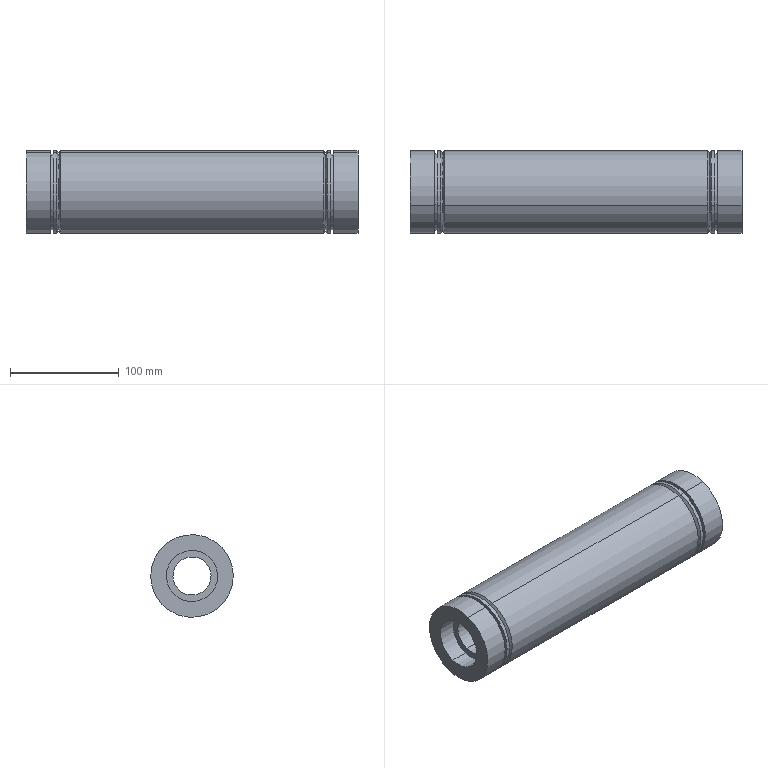Component | SolidWorks | DrivenRoller-1 | 3 solids | 50 faces | box 305 x 76 x 76 mm | volume 436807 mm3 | cylinder 28 | plane 14 | cone 8 | commonest cylinder face diameters 76 x10 68 x6 47 x4 35 x4 70 x4
build123d program:
from build123d import *
from OCP.BRepFilletAPI import BRepFilletAPI_MakeChamfer

# Parameters (mm, degrees)
SKETCH1_W      = 245
SKETCH1_H      = 4
CHAMFER1_SIZE  = 3
CHAMFER1_SIZE2 = 1.732
CHAMFER2_SIZE  = 3
CHAMFER2_SIZE2 = 1.732
CHAMFER3_SIZE  = 3
CHAMFER3_SIZE2 = 1.732


with BuildPart() as part:
    # Sketch1 → Revolve1 (revolve)
    with BuildSketch(Plane.XY, mode=Mode.PRIVATE) as revolve1_sk:
        with Locations((152.5, 36)):
            Rectangle(SKETCH1_W, SKETCH1_H)
    revolve(revolve1_sk.sketch.rotate(Axis((-4310.875, 0, 0), (1, 0, 0)), 90), axis=Axis((-4310.875, 0, 0), (1, 0, 0)))

    # Chamfer1: one chamfer whose edges measure the first distance from different faces: ONE call of the kernel's chamfer builder (chamfer() names one face for all edges)
    chamfer1_edges_1 = [part.edges().sort_by_distance(p)[0] for p in [
        (30, 0, -38),
    ]]
    chamfer1_side_1 = [part.faces().sort_by_distance(p)[0] for p in [
        (30, 0, -36.925),
    ]]
    chamfer1_edges_2 = [part.edges().sort_by_distance(p)[0] for p in [
        (275, 0, -38),
    ]]
    chamfer1_side_2 = [part.faces().sort_by_distance(p)[0] for p in [
        (275, 0, -35.075),
    ]]
    chamfer1 = BRepFilletAPI_MakeChamfer(part.part.solid().wrapped)
    for e in chamfer1_edges_1:
        chamfer1.Add(CHAMFER1_SIZE, CHAMFER1_SIZE2, e.wrapped, chamfer1_side_1[0].wrapped)  # the first distance lies on this face
    for e in chamfer1_edges_2:
        chamfer1.Add(CHAMFER1_SIZE, CHAMFER1_SIZE2, e.wrapped, chamfer1_side_2[0].wrapped)  # the first distance lies on this face
    add(Compound.cast(chamfer1.Shape()), mode=Mode.REPLACE)


with BuildPart() as body_2:
    # Sketch2 → Revolve2 (revolve)
    with BuildSketch(Plane.XY, mode=Mode.PRIVATE) as revolve2_sk:
        Polygon((0, 38), (22.5, 38), (22.5, 35), (25, 35), (25, 38), (30, 38), (30, 34), (36, 34), (36, 17.5), (16.5, 17.5), (16.5, 23.5), (0, 23.5), align=None)
        Polygon((275, 38), (280, 38), (280, 35), (282.5, 35), (282.5, 38), (305, 38), (305, 23.5), (288.5, 23.5), (288.5, 17.5), (269, 17.5), (269, 34), (275, 34), align=None)
    revolve(revolve2_sk.sketch.rotate(Axis((-1000, 0, 0), (1, 0, 0)), 90), axis=Axis((-1000, 0, 0), (1, 0, 0)))

    # Chamfer2
    chamfer2_edges = [body_2.edges().sort_by_distance(p)[0] for p in [
        (30, 0, -38),
    ]]
    chamfer2_side = [body_2.faces().sort_by_distance(p)[0] for p in [
        (30, 0, -36.925),
    ]]
    chamfer(chamfer2_edges, length=CHAMFER2_SIZE, length2=CHAMFER2_SIZE2, reference=chamfer2_side[0])

    # Chamfer3
    chamfer3_edges = [body_2.edges().sort_by_distance(p)[0] for p in [
        (275, 0, -38),
    ]]
    chamfer3_side = [body_2.faces().sort_by_distance(p)[0] for p in [
        (275, 0, -35.075),
    ]]
    chamfer(chamfer3_edges, length=CHAMFER3_SIZE, length2=CHAMFER3_SIZE2, reference=chamfer3_side[0])


solid = Compound([part.part, body_2.part])

# Placed as in the assembly
solid = solid.moved(Location((5782.506, 3057.679, 47.375), (0, 0, 0)))